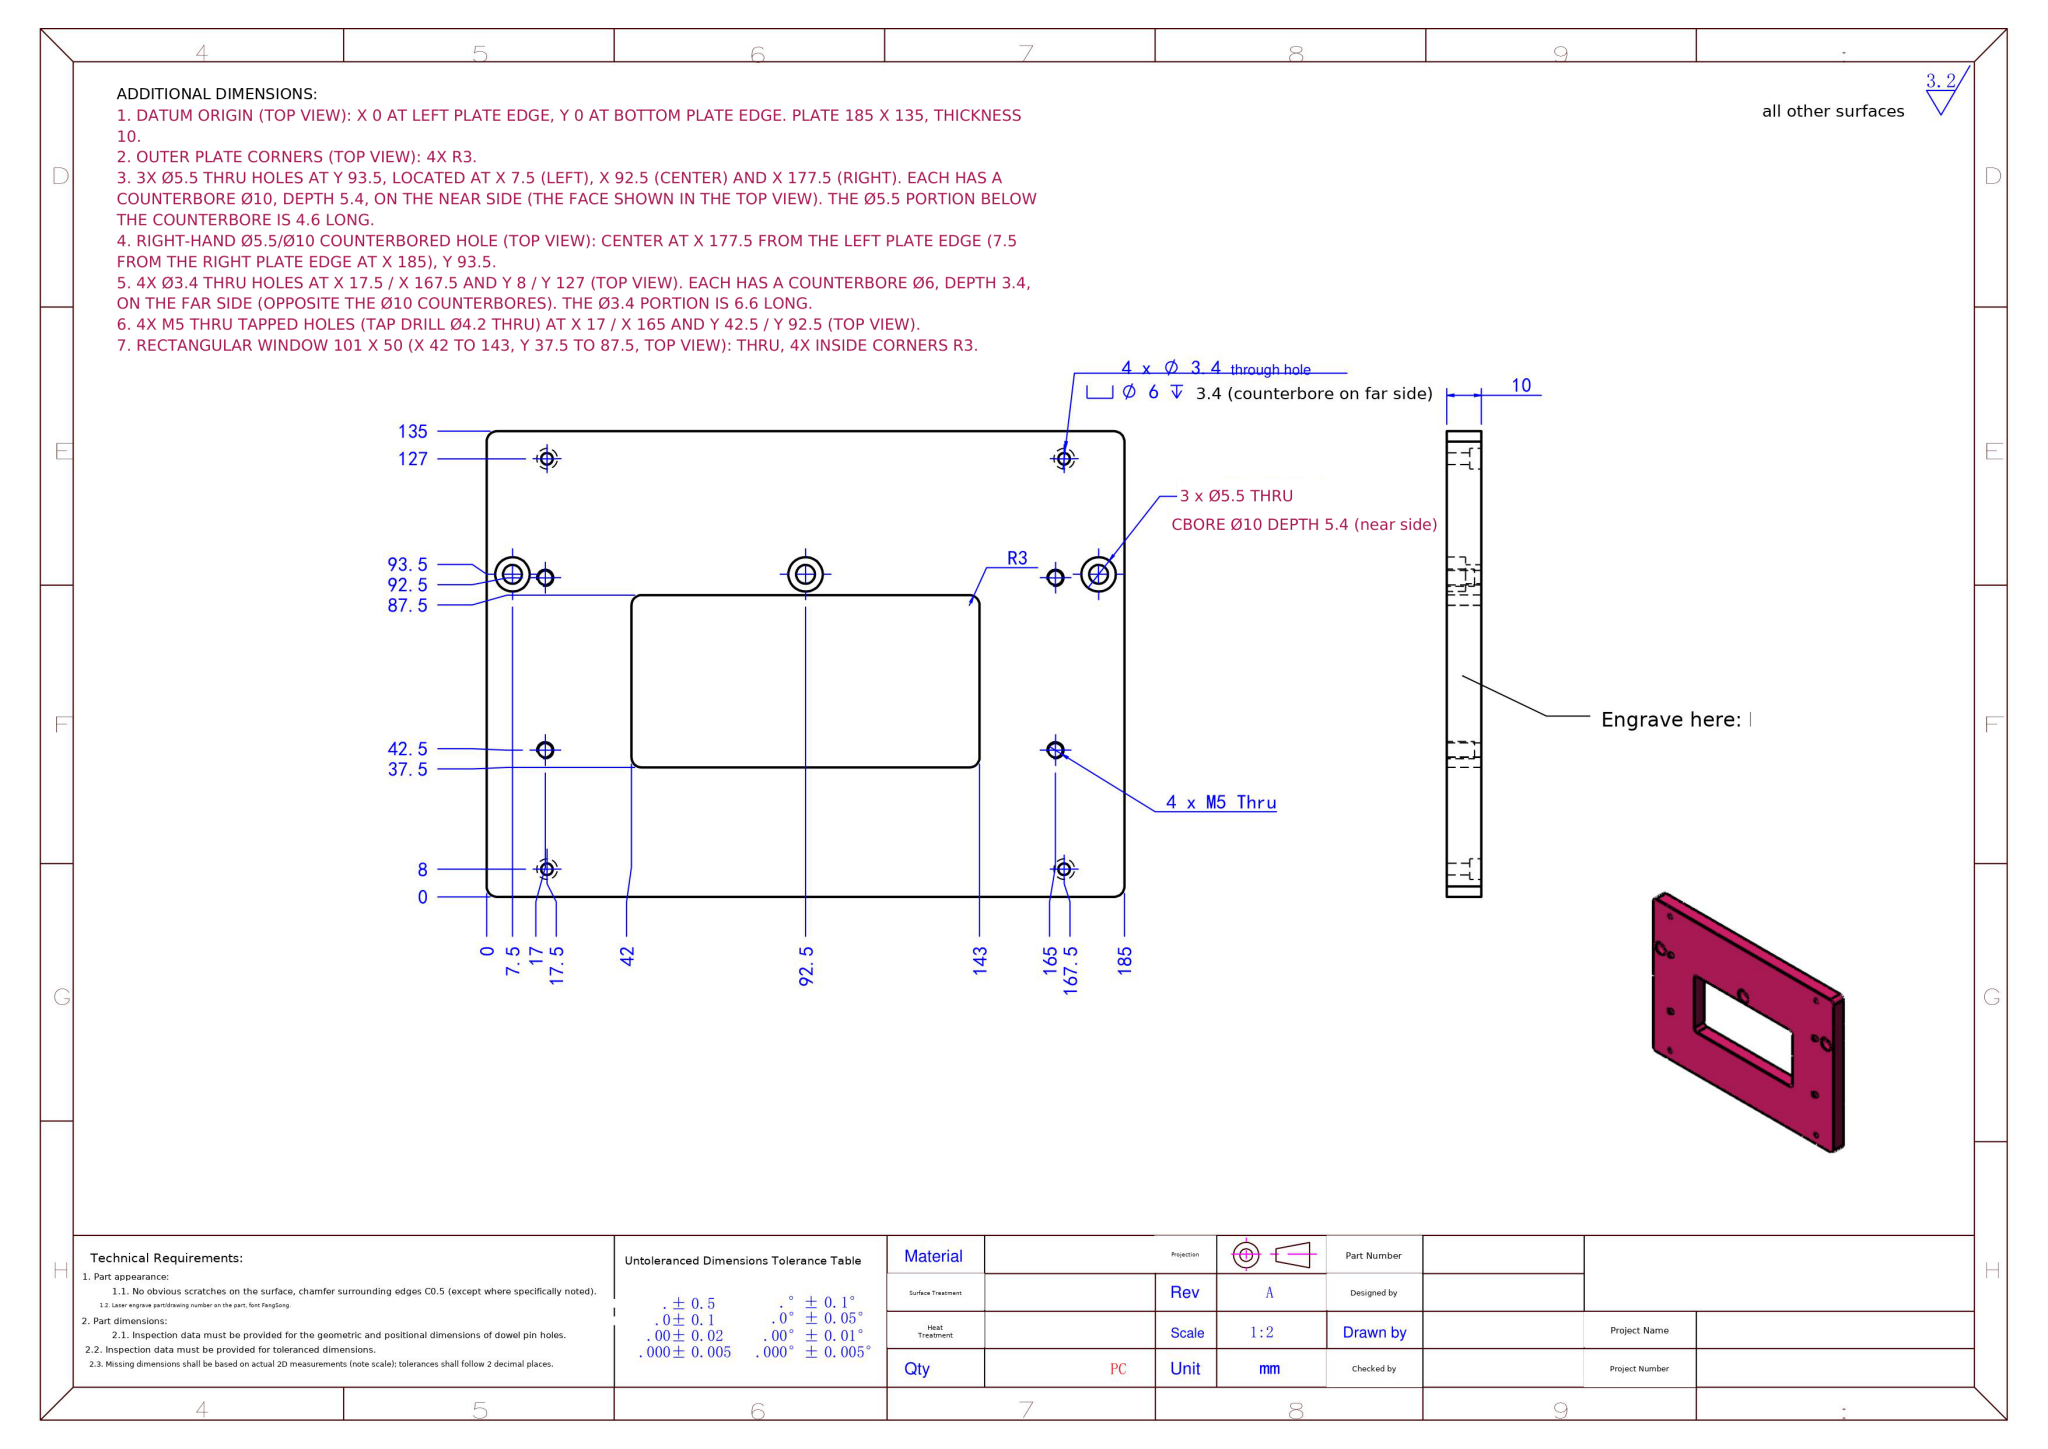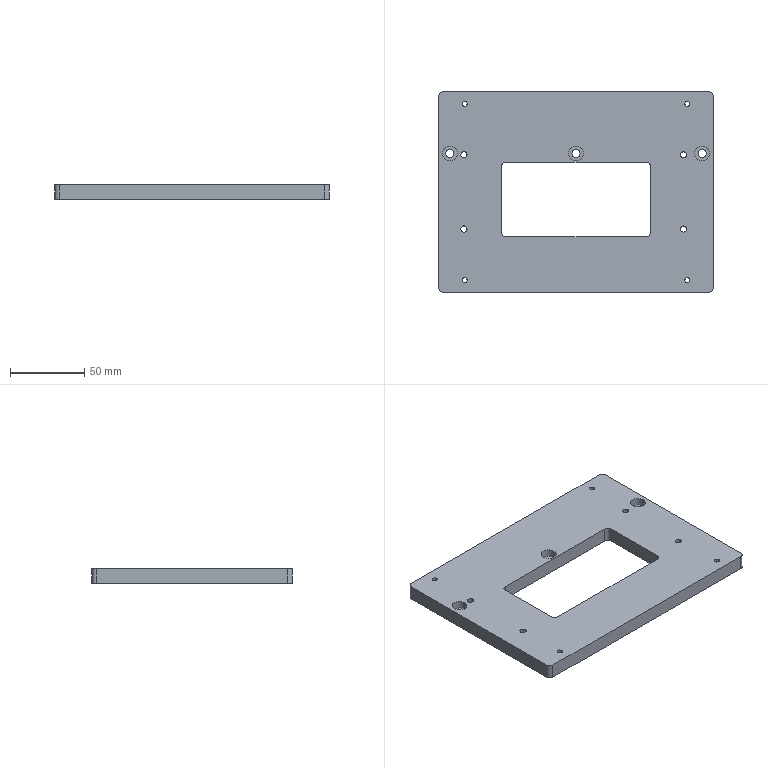Part | NX | mm | 1 solid | 61 faces | box 185 x 135 x 10 mm | volume 196471 mm3 | cylinder 44 | plane 17 | commonest cylinder face diameters 6 x16 3.4 x8 4.2 x8 10 x6 5.5 x6